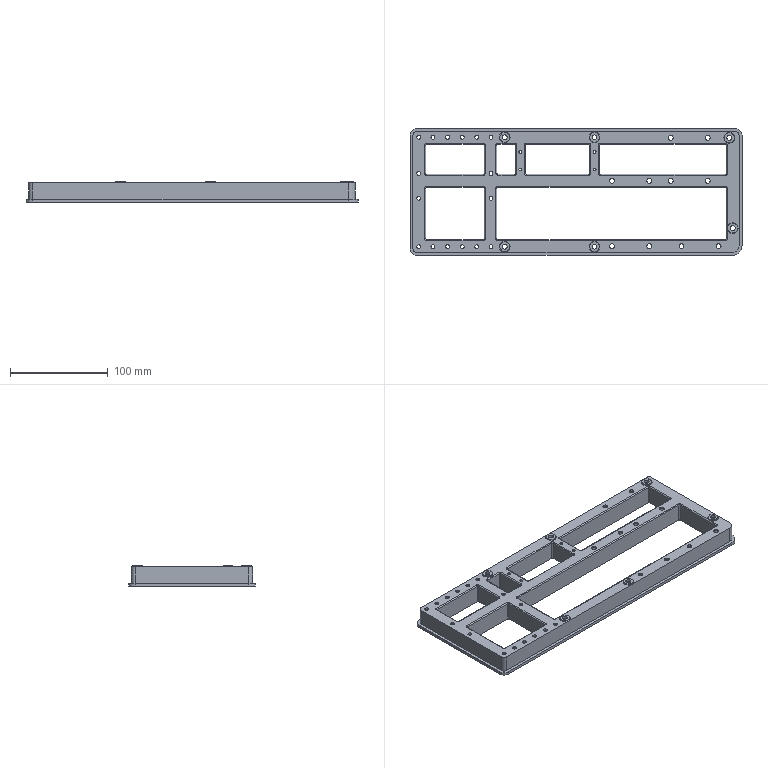Component | NX | BASE | 1 solid | 241 faces | volume 98865 mm3 | cylinder 130 | plane 81 | torus 30 | commonest cylinder face diameters 2 x48 5 x43 4 x16 10 x6 14 x4 11 x4 3 x4 8 x3